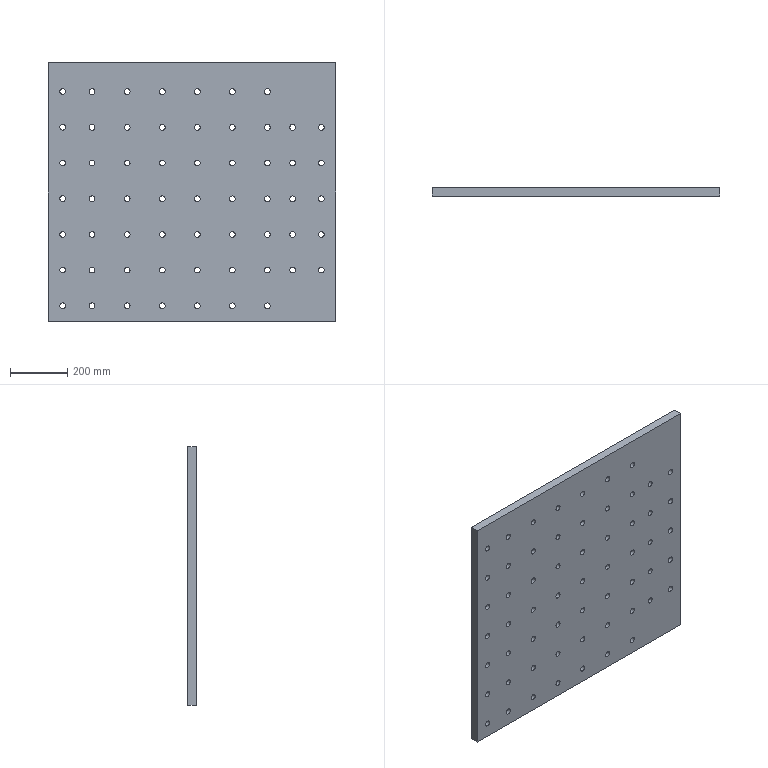Component | SolidWorks | MountingPlate-1 | 1 solid | 136 faces | box 1000 x 30 x 900 mm | volume 26418805 mm3 | cylinder 126 | plane 10 | commonest cylinder face diameters 20 x126 | material 45
build123d program:
from build123d import *

# Parameters (mm, degrees)
SKETCH1_W           = 1000
SKETCH1_H           = 900
BOSS_EXTRUDE1_DEPTH = 30
SKETCH2_R           = 10
CUT_EXTRUDE1_DEPTH  = 20
SKETCH4_R           = 10
CUT_EXTRUDE2_DEPTH  = 2919.122
SKETCH5_R           = 10
CUT_EXTRUDE3_DEPTH  = 2919.122
SKETCH7_R           = 10
CUT_EXTRUDE4_DEPTH  = 2919.122


with BuildPart() as part:
    # Sketch1 → Boss-Extrude1 (new body)
    with BuildSketch(Plane.XY):
        with Locations((2231.911, -575.281)):
            Rectangle(SKETCH1_W, SKETCH1_H)
    extrude(amount=BOSS_EXTRUDE1_DEPTH)

    # Sketch2 → Cut-Extrude1 (cut)
    with BuildSketch(Plane.XY.offset(30)):
        with Locations((2581.911, -179.241)):
            Circle(SKETCH2_R)
        with Locations((2681.911, -179.241)):
            Circle(SKETCH2_R)
        with Locations(Location((2681.911, -923.98, 0), (0, 0, 180))):
            Circle(SKETCH2_R)
        with Locations(Location((2581.911, -923.98, 0), (0, 0, 180))):
            Circle(SKETCH2_R)
    extrude(amount=-CUT_EXTRUDE1_DEPTH, mode=Mode.SUBTRACT)

    # Sketch4 → Cut-Extrude2 (cut, through all)
    with BuildSketch(Plane.XY.offset(30)):
        with Locations((1781.911, -179.241)):
            Circle(SKETCH4_R)
        with Locations((1884.348, -179.241)):
            Circle(SKETCH4_R)
        with Locations((2006.348, -179.241)):
            Circle(SKETCH4_R)
        with Locations((2128.348, -179.241)):
            Circle(SKETCH4_R)
        with Locations((2250.348, -179.241)):
            Circle(SKETCH4_R)
        with Locations((2372.348, -179.241)):
            Circle(SKETCH4_R)
        with Locations((2494.348, -179.241)):
            Circle(SKETCH4_R)
        with Locations((2006.348, -303.441)):
            Circle(SKETCH4_R)
        with Locations((2128.348, -303.441)):
            Circle(SKETCH4_R)
        with Locations((2250.348, -303.441)):
            Circle(SKETCH4_R)
        with Locations((2372.348, -303.441)):
            Circle(SKETCH4_R)
        with Locations((2494.348, -303.441)):
            Circle(SKETCH4_R)
        with Locations((2006.348, -427.641)):
            Circle(SKETCH4_R)
        with Locations((2128.348, -427.641)):
            Circle(SKETCH4_R)
        with Locations((2250.348, -427.641)):
            Circle(SKETCH4_R)
        with Locations((2372.348, -427.641)):
            Circle(SKETCH4_R)
        with Locations((2494.348, -427.641)):
            Circle(SKETCH4_R)
        with Locations((2006.348, -551.841)):
            Circle(SKETCH4_R)
        with Locations((2128.348, -551.841)):
            Circle(SKETCH4_R)
        with Locations((2250.348, -551.841)):
            Circle(SKETCH4_R)
        with Locations((2372.348, -551.841)):
            Circle(SKETCH4_R)
        with Locations((2494.348, -551.841)):
            Circle(SKETCH4_R)
        with Locations((2006.348, -676.041)):
            Circle(SKETCH4_R)
        with Locations((2128.348, -676.041)):
            Circle(SKETCH4_R)
        with Locations((2250.348, -676.041)):
            Circle(SKETCH4_R)
        with Locations((2372.348, -676.041)):
            Circle(SKETCH4_R)
        with Locations((2494.348, -676.041)):
            Circle(SKETCH4_R)
        with Locations((2006.348, -800.241)):
            Circle(SKETCH4_R)
        with Locations((2128.348, -800.241)):
            Circle(SKETCH4_R)
        with Locations((2250.348, -800.241)):
            Circle(SKETCH4_R)
        with Locations((2372.348, -800.241)):
            Circle(SKETCH4_R)
        with Locations((2494.348, -800.241)):
            Circle(SKETCH4_R)
        with Locations((2006.348, -924.441)):
            Circle(SKETCH4_R)
        with Locations((2128.348, -924.441)):
            Circle(SKETCH4_R)
        with Locations((2250.348, -924.441)):
            Circle(SKETCH4_R)
        with Locations((2372.348, -924.441)):
            Circle(SKETCH4_R)
        with Locations((2494.348, -924.441)):
            Circle(SKETCH4_R)
        with Locations((1884.348, -303.441)):
            Circle(SKETCH4_R)
        with Locations((1884.348, -427.641)):
            Circle(SKETCH4_R)
        with Locations((1884.348, -551.841)):
            Circle(SKETCH4_R)
        with Locations((1884.348, -676.041)):
            Circle(SKETCH4_R)
        with Locations((1884.348, -800.241)):
            Circle(SKETCH4_R)
        with Locations((1884.348, -924.441)):
            Circle(SKETCH4_R)
    extrude(amount=-CUT_EXTRUDE2_DEPTH, mode=Mode.SUBTRACT)

    # Sketch5 → Cut-Extrude3 (cut, through all)
    with BuildSketch(Plane.XY.offset(30)):
        with Locations((1781.911, -179.241)):
            Circle(SKETCH5_R)
        with Locations((1781.911, -303.541)):
            Circle(SKETCH5_R)
        with Locations((1781.911, -427.841)):
            Circle(SKETCH5_R)
        with Locations((1781.911, -552.141)):
            Circle(SKETCH5_R)
        with Locations((1781.911, -676.441)):
            Circle(SKETCH5_R)
        with Locations((1781.911, -800.741)):
            Circle(SKETCH5_R)
        with Locations((1781.911, -925.041)):
            Circle(SKETCH5_R)
    extrude(amount=-CUT_EXTRUDE3_DEPTH, mode=Mode.SUBTRACT)

    # Sketch7 → Cut-Extrude4 (cut, through all)
    with BuildSketch(Plane.XY.offset(30)):
        with Locations((2581.911, -303.441)):
            Circle(SKETCH7_R)
        with Locations((2681.911, -303.441)):
            Circle(SKETCH7_R)
        with Locations((2681.911, -427.641)):
            Circle(SKETCH7_R)
        with Locations((2581.911, -427.641)):
            Circle(SKETCH7_R)
        with Locations((2681.911, -551.841)):
            Circle(SKETCH7_R)
        with Locations((2581.911, -551.841)):
            Circle(SKETCH7_R)
        with Locations((2681.911, -676.041)):
            Circle(SKETCH7_R)
        with Locations((2581.911, -676.041)):
            Circle(SKETCH7_R)
        with Locations((2681.911, -800.241)):
            Circle(SKETCH7_R)
        with Locations((2581.911, -800.241)):
            Circle(SKETCH7_R)
    extrude(amount=-CUT_EXTRUDE4_DEPTH, mode=Mode.SUBTRACT)


solid = part.part

# Placed as in the assembly
solid = solid.moved(Location((-545.911, -831, -80.281), (-90, 0, 0)))